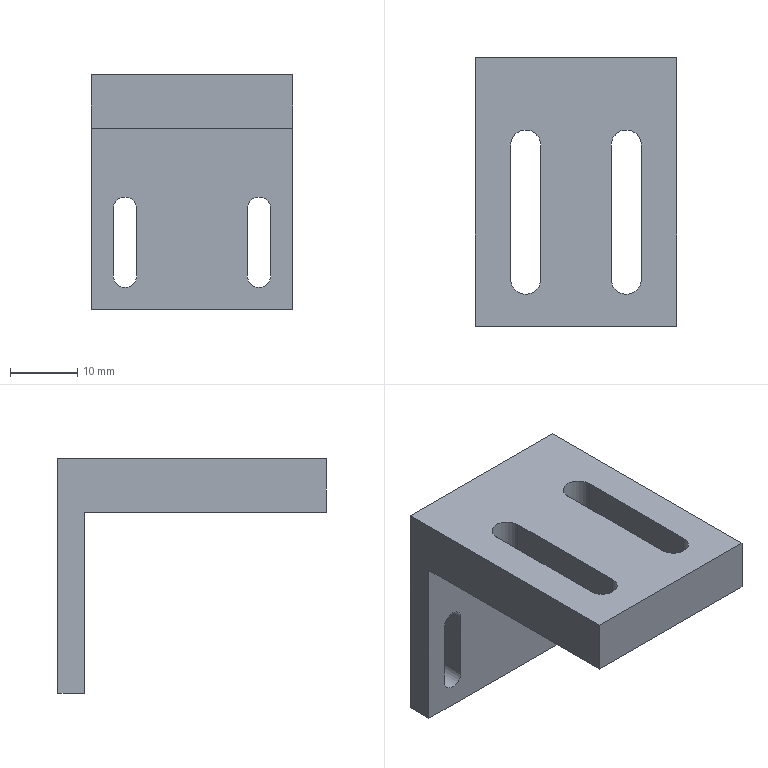Component | SolidWorks | CS021-A10-A028-1 | 1 solid | 26 faces | box 30 x 40 x 35 mm | volume 10789 mm3 | plane 16 | cylinder 10 | commonest cylinder face diameters 3.5 x6 4.5 x4 | material AL6061
build123d program:
from build123d import *

# Parameters (mm, degrees)
BOSS_EXTRUDE1_DEPTH = 15
CUT_EXTRUDE1_DEPTH  = 56.227
CUT_EXTRUDE2_DEPTH  = 56.227


with BuildPart() as part:
    # Sketch1 → Boss-Extrude1 (new, symmetric)
    with BuildSketch(Plane.XY):
        Polygon((0, 0), (8, 0), (8, 36), (35, 36), (35, 40), (0, 40), align=None)
    extrude(amount=BOSS_EXTRUDE1_DEPTH, both=True)

    # Sketch2 → Cut-Extrude1 (cut, through all)
    with BuildSketch(Plane.ZY):
        with BuildLine():
            Line((-9.75, 7), (-9.75, 27))
            ThreePointArc((-9.75, 27), (-7.5, 29.25), (-5.25, 27))
            Line((-5.25, 27), (-5.25, 7))
            ThreePointArc((-5.25, 7), (-7.5, 4.75), (-9.75, 7))
        make_face()
        with BuildLine():
            Line((9.75, 7), (9.75, 27))
            ThreePointArc((9.75, 27), (7.5, 29.25), (5.25, 27))
            Line((5.25, 27), (5.25, 7))
            ThreePointArc((5.25, 7), (7.5, 4.75), (9.75, 7))
        make_face()
    extrude(amount=-CUT_EXTRUDE1_DEPTH, mode=Mode.SUBTRACT)

    # Sketch3 → Cut-Extrude2 (cut, through all)
    with BuildSketch(Plane(origin=(0, 40, 0), x_dir=(1, 0, 0), z_dir=(0, 1, 0))):
        with BuildLine():
            Line((20, 11.75), (30, 11.75))
            ThreePointArc((30, 11.75), (31.75, 10), (30, 8.25))
            Line((30, 8.25), (20, 8.25))
            ThreePointArc((20, 8.25), (18.25, 10), (20, 11.75))
        make_face()
        with BuildLine():
            Line((20, -11.75), (30, -11.75))
            ThreePointArc((30, -11.75), (31.75, -10), (30, -8.25))
            Line((30, -8.25), (20, -8.25))
            ThreePointArc((20, -8.25), (18.25, -10), (20, -11.75))
        make_face()
    extrude(amount=-CUT_EXTRUDE2_DEPTH, mode=Mode.SUBTRACT)


solid = part.part

# Placed as in the assembly
solid = solid.moved(Location((152.449, 58.817, -55), (0, 90, 0)))
STEP:
#1=COLOUR_RGB('',0.7922,0.8196,0.9333);
#2=FILL_AREA_STYLE_COLOUR('',#1);
#3=FILL_AREA_STYLE('',(#2));
#4=SURFACE_STYLE_FILL_AREA(#3);
#5=SURFACE_SIDE_STYLE('',(#4));
#6=SURFACE_STYLE_USAGE(.BOTH.,#5);
#7=PRESENTATION_STYLE_ASSIGNMENT((#6));
#8=CARTESIAN_POINT('',(6.396,3.733,-2.884));
#9=VERTEX_POINT('',#8);
#10=CARTESIAN_POINT('',(6.465,3.733,-2.953));
#11=VERTEX_POINT('',#10);
#12=CARTESIAN_POINT('',(6.396,3.733,-2.953));
#13=DIRECTION('',(0.,1.,-0.));
#14=DIRECTION('',(1.,0.,0.));
#15=AXIS2_PLACEMENT_3D('',#12,#13,#14);
#16=CIRCLE('',#15,0.0689);
#17=EDGE_CURVE('',#9,#11,#16,.T.);
#18=ORIENTED_EDGE('',*,*,#17,.F.);
#19=CARTESIAN_POINT('',(6.396,3.89,-2.884));
#20=VERTEX_POINT('',#19);
#21=CARTESIAN_POINT('',(6.396,2.316,-2.884));
#22=DIRECTION('',(0.,1.,0.));
#23=VECTOR('',#22,39.37);
#24=LINE('',#21,#23);
#25=EDGE_CURVE('',#9,#20,#24,.T.);
#26=ORIENTED_EDGE('',*,*,#25,.T.);
#27=CARTESIAN_POINT('',(6.465,3.89,-2.953));
#28=VERTEX_POINT('',#27);
#29=CARTESIAN_POINT('',(6.396,3.89,-2.953));
#30=DIRECTION('',(0.,1.,0.));
#31=DIRECTION('',(0.,0.,-1.));
#32=AXIS2_PLACEMENT_3D('',#29,#30,#31);
#33=CIRCLE('',#32,0.0689);
#34=EDGE_CURVE('',#20,#28,#33,.T.);
#35=ORIENTED_EDGE('',*,*,#34,.T.);
#36=CARTESIAN_POINT('',(6.465,2.316,-2.953));
#37=DIRECTION('',(0.,1.,0.));
#38=VECTOR('',#37,39.37);
#39=LINE('',#36,#38);
#40=EDGE_CURVE('',#11,#28,#39,.T.);
#41=ORIENTED_EDGE('',*,*,#40,.F.);
#42=EDGE_LOOP('',(#18,#26,#35,#41));
#43=FACE_OUTER_BOUND('',#42,.T.);
#44=CARTESIAN_POINT('',(6.396,2.316,-2.953));
#45=DIRECTION('',(0.,1.,0.));
#46=DIRECTION('',(0.,0.,1.));
#47=AXIS2_PLACEMENT_3D('',#44,#45,#46);
#48=CYLINDRICAL_SURFACE('',#47,0.0689);
#49=ADVANCED_FACE('',(#43),#48,.F.);
#50=CARTESIAN_POINT('',(5.608,3.733,-2.884));
#51=VERTEX_POINT('',#50);
#52=CARTESIAN_POINT('',(5.677,3.733,-2.953));
#53=VERTEX_POINT('',#52);
#54=CARTESIAN_POINT('',(5.608,3.733,-2.953));
#55=DIRECTION('',(0.,1.,-0.));
#56=DIRECTION('',(1.,0.,0.));
#57=AXIS2_PLACEMENT_3D('',#54,#55,#56);
#58=CIRCLE('',#57,0.0689);
#59=EDGE_CURVE('',#51,#53,#58,.T.);
#60=ORIENTED_EDGE('',*,*,#59,.F.);
#61=CARTESIAN_POINT('',(5.608,3.89,-2.884));
#62=VERTEX_POINT('',#61);
#63=CARTESIAN_POINT('',(5.608,2.316,-2.884));
#64=DIRECTION('',(0.,1.,0.));
#65=VECTOR('',#64,39.37);
#66=LINE('',#63,#65);
#67=EDGE_CURVE('',#51,#62,#66,.T.);
#68=ORIENTED_EDGE('',*,*,#67,.T.);
#69=CARTESIAN_POINT('',(5.677,3.89,-2.953));
#70=VERTEX_POINT('',#69);
#71=CARTESIAN_POINT('',(5.608,3.89,-2.953));
#72=DIRECTION('',(0.,1.,0.));
#73=DIRECTION('',(0.,0.,1.));
#74=AXIS2_PLACEMENT_3D('',#71,#72,#73);
#75=CIRCLE('',#74,0.0689);
#76=EDGE_CURVE('',#62,#70,#75,.T.);
#77=ORIENTED_EDGE('',*,*,#76,.T.);
#78=CARTESIAN_POINT('',(5.677,2.316,-2.953));
#79=DIRECTION('',(0.,1.,0.));
#80=VECTOR('',#79,39.37);
#81=LINE('',#78,#80);
#82=EDGE_CURVE('',#53,#70,#81,.T.);
#83=ORIENTED_EDGE('',*,*,#82,.F.);
#84=EDGE_LOOP('',(#60,#68,#77,#83));
#85=FACE_OUTER_BOUND('',#84,.T.);
#86=CARTESIAN_POINT('',(5.608,2.316,-2.953));
#87=DIRECTION('',(0.,1.,0.));
#88=DIRECTION('',(0.,0.,1.));
#89=AXIS2_PLACEMENT_3D('',#86,#87,#88);
#90=CYLINDRICAL_SURFACE('',#89,0.0689);
#91=ADVANCED_FACE('',(#85),#90,.F.);
#92=CARTESIAN_POINT('',(6.386,2.591,-2.165));
#93=VERTEX_POINT('',#92);
#94=CARTESIAN_POINT('',(6.386,3.379,-2.165));
#95=VERTEX_POINT('',#94);
#96=CARTESIAN_POINT('',(6.386,2.591,-2.165));
#97=DIRECTION('',(0.,1.,-0.));
#98=VECTOR('',#97,39.37);
#99=LINE('',#96,#98);
#100=EDGE_CURVE('',#93,#95,#99,.T.);
#101=ORIENTED_EDGE('',*,*,#100,.F.);
#102=CARTESIAN_POINT('',(6.209,2.591,-2.165));
#103=VERTEX_POINT('',#102);
#104=CARTESIAN_POINT('',(6.297,2.591,-2.165));
#105=DIRECTION('',(0.,0.,1.));
#106=DIRECTION('',(-1.,0.,0.));
#107=AXIS2_PLACEMENT_3D('',#104,#105,#106);
#108=CIRCLE('',#107,0.08858);
#109=EDGE_CURVE('',#103,#93,#108,.T.);
#110=ORIENTED_EDGE('',*,*,#109,.F.);
#111=CARTESIAN_POINT('',(6.209,3.379,-2.165));
#112=VERTEX_POINT('',#111);
#113=CARTESIAN_POINT('',(6.209,2.591,-2.165));
#114=DIRECTION('',(-0.,-1.,0.));
#115=VECTOR('',#114,39.37);
#116=LINE('',#113,#115);
#117=EDGE_CURVE('',#112,#103,#116,.T.);
#118=ORIENTED_EDGE('',*,*,#117,.F.);
#119=CARTESIAN_POINT('',(6.297,3.379,-2.165));
#120=DIRECTION('',(0.,0.,1.));
#121=DIRECTION('',(-1.,0.,0.));
#122=AXIS2_PLACEMENT_3D('',#119,#120,#121);
#123=CIRCLE('',#122,0.08858);
#124=EDGE_CURVE('',#95,#112,#123,.T.);
#125=ORIENTED_EDGE('',*,*,#124,.F.);
#126=EDGE_LOOP('',(#101,#110,#118,#125));
#127=FACE_BOUND('',#126,.T.);
#128=CARTESIAN_POINT('',(5.795,2.591,-2.165));
#129=VERTEX_POINT('',#128);
#130=CARTESIAN_POINT('',(5.795,3.379,-2.165));
#131=VERTEX_POINT('',#130);
#132=CARTESIAN_POINT('',(5.795,2.591,-2.165));
#133=DIRECTION('',(0.,1.,-0.));
#134=VECTOR('',#133,39.37);
#135=LINE('',#132,#134);
#136=EDGE_CURVE('',#129,#131,#135,.T.);
#137=ORIENTED_EDGE('',*,*,#136,.F.);
#138=CARTESIAN_POINT('',(5.618,2.591,-2.165));
#139=VERTEX_POINT('',#138);
#140=CARTESIAN_POINT('',(5.707,2.591,-2.165));
#141=DIRECTION('',(0.,0.,1.));
#142=DIRECTION('',(1.,0.,0.));
#143=AXIS2_PLACEMENT_3D('',#140,#141,#142);
#144=CIRCLE('',#143,0.08858);
#145=EDGE_CURVE('',#139,#129,#144,.T.);
#146=ORIENTED_EDGE('',*,*,#145,.F.);
#147=CARTESIAN_POINT('',(5.618,3.379,-2.165));
#148=VERTEX_POINT('',#147);
#149=CARTESIAN_POINT('',(5.618,2.591,-2.165));
#150=DIRECTION('',(-0.,-1.,0.));
#151=VECTOR('',#150,39.37);
#152=LINE('',#149,#151);
#153=EDGE_CURVE('',#148,#139,#152,.T.);
#154=ORIENTED_EDGE('',*,*,#153,.F.);
#155=CARTESIAN_POINT('',(5.707,3.379,-2.165));
#156=DIRECTION('',(0.,0.,1.));
#157=DIRECTION('',(1.,0.,0.));
#158=AXIS2_PLACEMENT_3D('',#155,#156,#157);
#159=CIRCLE('',#158,0.08858);
#160=EDGE_CURVE('',#131,#148,#159,.T.);
#161=ORIENTED_EDGE('',*,*,#160,.F.);
#162=EDGE_LOOP('',(#137,#146,#154,#161));
#163=FACE_BOUND('',#162,.T.);
#164=CARTESIAN_POINT('',(5.411,3.89,-2.165));
#165=VERTEX_POINT('',#164);
#166=CARTESIAN_POINT('',(5.411,2.316,-2.165));
#167=VERTEX_POINT('',#166);
#168=CARTESIAN_POINT('',(5.411,3.89,-2.165));
#169=DIRECTION('',(-0.,-1.,0.));
#170=VECTOR('',#169,39.37);
#171=LINE('',#168,#170);
#172=EDGE_CURVE('',#165,#167,#171,.T.);
#173=ORIENTED_EDGE('',*,*,#172,.T.);
#174=CARTESIAN_POINT('',(6.592,2.316,-2.165));
#175=VERTEX_POINT('',#174);
#176=CARTESIAN_POINT('',(6.592,2.316,-2.165));
#177=DIRECTION('',(-1.,0.,0.));
#178=VECTOR('',#177,39.37);
#179=LINE('',#176,#178);
#180=EDGE_CURVE('',#175,#167,#179,.T.);
#181=ORIENTED_EDGE('',*,*,#180,.F.);
#182=CARTESIAN_POINT('',(6.592,3.89,-2.165));
#183=VERTEX_POINT('',#182);
#184=CARTESIAN_POINT('',(6.592,3.89,-2.165));
#185=DIRECTION('',(-0.,-1.,0.));
#186=VECTOR('',#185,39.37);
#187=LINE('',#184,#186);
#188=EDGE_CURVE('',#183,#175,#187,.T.);
#189=ORIENTED_EDGE('',*,*,#188,.F.);
#190=CARTESIAN_POINT('',(6.592,3.89,-2.165));
#191=DIRECTION('',(-1.,0.,0.));
#192=VECTOR('',#191,39.37);
#193=LINE('',#190,#192);
#194=EDGE_CURVE('',#183,#165,#193,.T.);
#195=ORIENTED_EDGE('',*,*,#194,.T.);
#196=EDGE_LOOP('',(#173,#181,#189,#195));
#197=FACE_OUTER_BOUND('',#196,.T.);
#198=CARTESIAN_POINT('',(6.592,3.89,-2.165));
#199=DIRECTION('',(-0.,-0.,-1.));
#200=DIRECTION('',(-1.,0.,0.));
#201=AXIS2_PLACEMENT_3D('',#198,#199,#200);
#202=PLANE('',#201);
#203=ADVANCED_FACE('',(#127,#163,#197),#202,.F.);
#204=CARTESIAN_POINT('',(5.411,2.316,-2.48));
#205=VERTEX_POINT('',#204);
#206=CARTESIAN_POINT('',(5.411,2.316,-2.165));
#207=DIRECTION('',(-0.,-0.,-1.));
#208=VECTOR('',#207,39.37);
#209=LINE('',#206,#208);
#210=EDGE_CURVE('',#167,#205,#209,.T.);
#211=ORIENTED_EDGE('',*,*,#210,.T.);
#212=CARTESIAN_POINT('',(6.592,2.316,-2.48));
#213=VERTEX_POINT('',#212);
#214=CARTESIAN_POINT('',(6.592,2.316,-2.48));
#215=DIRECTION('',(-1.,0.,0.));
#216=VECTOR('',#215,39.37);
#217=LINE('',#214,#216);
#218=EDGE_CURVE('',#213,#205,#217,.T.);
#219=ORIENTED_EDGE('',*,*,#218,.F.);
#220=CARTESIAN_POINT('',(6.592,2.316,-2.165));
#221=DIRECTION('',(-0.,-0.,-1.));
#222=VECTOR('',#221,39.37);
#223=LINE('',#220,#222);
#224=EDGE_CURVE('',#175,#213,#223,.T.);
#225=ORIENTED_EDGE('',*,*,#224,.F.);
#226=ORIENTED_EDGE('',*,*,#180,.T.);
#227=EDGE_LOOP('',(#211,#219,#225,#226));
#228=FACE_OUTER_BOUND('',#227,.T.);
#229=CARTESIAN_POINT('',(6.592,2.316,-2.165));
#230=DIRECTION('',(0.,1.,-0.));
#231=DIRECTION('',(1.,-0.,-0.));
#232=AXIS2_PLACEMENT_3D('',#229,#230,#231);
#233=PLANE('',#232);
#234=ADVANCED_FACE('',(#228),#233,.F.);
#235=CARTESIAN_POINT('',(6.209,3.379,-2.48));
#236=VERTEX_POINT('',#235);
#237=CARTESIAN_POINT('',(6.209,2.591,-2.48));
#238=VERTEX_POINT('',#237);
#239=CARTESIAN_POINT('',(6.209,2.316,-2.48));
#240=DIRECTION('',(-0.,-1.,0.));
#241=VECTOR('',#240,39.37);
#242=LINE('',#239,#241);
#243=EDGE_CURVE('',#236,#238,#242,.T.);
#244=ORIENTED_EDGE('',*,*,#243,.T.);
#245=CARTESIAN_POINT('',(6.386,2.591,-2.48));
#246=VERTEX_POINT('',#245);
#247=CARTESIAN_POINT('',(6.297,2.591,-2.48));
#248=DIRECTION('',(0.,0.,1.));
#249=DIRECTION('',(1.,0.,0.));
#250=AXIS2_PLACEMENT_3D('',#247,#248,#249);
#251=CIRCLE('',#250,0.08858);
#252=EDGE_CURVE('',#238,#246,#251,.T.);
#253=ORIENTED_EDGE('',*,*,#252,.T.);
#254=CARTESIAN_POINT('',(6.386,3.379,-2.48));
#255=VERTEX_POINT('',#254);
#256=CARTESIAN_POINT('',(6.386,2.316,-2.48));
#257=DIRECTION('',(0.,1.,-0.));
#258=VECTOR('',#257,39.37);
#259=LINE('',#256,#258);
#260=EDGE_CURVE('',#246,#255,#259,.T.);
#261=ORIENTED_EDGE('',*,*,#260,.T.);
#262=CARTESIAN_POINT('',(6.297,3.379,-2.48));
#263=DIRECTION('',(0.,0.,1.));
#264=DIRECTION('',(1.,0.,0.));
#265=AXIS2_PLACEMENT_3D('',#262,#263,#264);
#266=CIRCLE('',#265,0.08858);
#267=EDGE_CURVE('',#255,#236,#266,.T.);
#268=ORIENTED_EDGE('',*,*,#267,.T.);
#269=EDGE_LOOP('',(#244,#253,#261,#268));
#270=FACE_BOUND('',#269,.T.);
#271=CARTESIAN_POINT('',(5.618,3.379,-2.48));
#272=VERTEX_POINT('',#271);
#273=CARTESIAN_POINT('',(5.618,2.591,-2.48));
#274=VERTEX_POINT('',#273);
#275=CARTESIAN_POINT('',(5.618,2.316,-2.48));
#276=DIRECTION('',(-0.,-1.,0.));
#277=VECTOR('',#276,39.37);
#278=LINE('',#275,#277);
#279=EDGE_CURVE('',#272,#274,#278,.T.);
#280=ORIENTED_EDGE('',*,*,#279,.T.);
#281=CARTESIAN_POINT('',(5.795,2.591,-2.48));
#282=VERTEX_POINT('',#281);
#283=CARTESIAN_POINT('',(5.707,2.591,-2.48));
#284=DIRECTION('',(0.,0.,1.));
#285=DIRECTION('',(1.,0.,0.));
#286=AXIS2_PLACEMENT_3D('',#283,#284,#285);
#287=CIRCLE('',#286,0.08858);
#288=EDGE_CURVE('',#274,#282,#287,.T.);
#289=ORIENTED_EDGE('',*,*,#288,.T.);
#290=CARTESIAN_POINT('',(5.795,3.379,-2.48));
#291=VERTEX_POINT('',#290);
#292=CARTESIAN_POINT('',(5.795,2.316,-2.48));
#293=DIRECTION('',(0.,1.,-0.));
#294=VECTOR('',#293,39.37);
#295=LINE('',#292,#294);
#296=EDGE_CURVE('',#282,#291,#295,.T.);
#297=ORIENTED_EDGE('',*,*,#296,.T.);
#298=CARTESIAN_POINT('',(5.707,3.379,-2.48));
#299=DIRECTION('',(0.,0.,1.));
#300=DIRECTION('',(1.,0.,0.));
#301=AXIS2_PLACEMENT_3D('',#298,#299,#300);
#302=CIRCLE('',#301,0.08858);
#303=EDGE_CURVE('',#291,#272,#302,.T.);
#304=ORIENTED_EDGE('',*,*,#303,.T.);
#305=EDGE_LOOP('',(#280,#289,#297,#304));
#306=FACE_BOUND('',#305,.T.);
#307=CARTESIAN_POINT('',(5.411,3.733,-2.48));
#308=VERTEX_POINT('',#307);
#309=CARTESIAN_POINT('',(5.411,2.316,-2.48));
#310=DIRECTION('',(0.,1.,-0.));
#311=VECTOR('',#310,39.37);
#312=LINE('',#309,#311);
#313=EDGE_CURVE('',#205,#308,#312,.T.);
#314=ORIENTED_EDGE('',*,*,#313,.T.);
#315=CARTESIAN_POINT('',(6.592,3.733,-2.48));
#316=VERTEX_POINT('',#315);
#317=CARTESIAN_POINT('',(6.592,3.733,-2.48));
#318=DIRECTION('',(-1.,0.,0.));
#319=VECTOR('',#318,39.37);
#320=LINE('',#317,#319);
#321=EDGE_CURVE('',#316,#308,#320,.T.);
#322=ORIENTED_EDGE('',*,*,#321,.F.);
#323=CARTESIAN_POINT('',(6.592,2.316,-2.48));
#324=DIRECTION('',(0.,1.,-0.));
#325=VECTOR('',#324,39.37);
#326=LINE('',#323,#325);
#327=EDGE_CURVE('',#213,#316,#326,.T.);
#328=ORIENTED_EDGE('',*,*,#327,.F.);
#329=ORIENTED_EDGE('',*,*,#218,.T.);
#330=EDGE_LOOP('',(#314,#322,#328,#329));
#331=FACE_OUTER_BOUND('',#330,.T.);
#332=CARTESIAN_POINT('',(6.592,2.316,-2.48));
#333=DIRECTION('',(0.,0.,1.));
#334=DIRECTION('',(1.,-0.,-0.));
#335=AXIS2_PLACEMENT_3D('',#332,#333,#334);
#336=PLANE('',#335);
#337=ADVANCED_FACE('',(#270,#306,#331),#336,.F.);
#338=CARTESIAN_POINT('',(6.327,3.733,-3.346));
#339=VERTEX_POINT('',#338);
#340=CARTESIAN_POINT('',(6.327,3.733,-2.953));
#341=VERTEX_POINT('',#340);
#342=CARTESIAN_POINT('',(6.327,3.733,-2.48));
#343=DIRECTION('',(0.,0.,1.));
#344=VECTOR('',#343,39.37);
#345=LINE('',#342,#344);
#346=EDGE_CURVE('',#339,#341,#345,.T.);
#347=ORIENTED_EDGE('',*,*,#346,.T.);
#348=CARTESIAN_POINT('',(6.396,3.733,-2.953));
#349=DIRECTION('',(0.,1.,-0.));
#350=DIRECTION('',(1.,0.,0.));
#351=AXIS2_PLACEMENT_3D('',#348,#349,#350);
#352=CIRCLE('',#351,0.0689);
#353=EDGE_CURVE('',#341,#9,#352,.T.);
#354=ORIENTED_EDGE('',*,*,#353,.T.);
#355=ORIENTED_EDGE('',*,*,#17,.T.);
#356=CARTESIAN_POINT('',(6.465,3.733,-3.346));
#357=VERTEX_POINT('',#356);
#358=CARTESIAN_POINT('',(6.465,3.733,-2.48));
#359=DIRECTION('',(-0.,-0.,-1.));
#360=VECTOR('',#359,39.37);
#361=LINE('',#358,#360);
#362=EDGE_CURVE('',#11,#357,#361,.T.);
#363=ORIENTED_EDGE('',*,*,#362,.T.);
#364=CARTESIAN_POINT('',(6.396,3.733,-3.346));
#365=DIRECTION('',(0.,1.,-0.));
#366=DIRECTION('',(1.,0.,0.));
#367=AXIS2_PLACEMENT_3D('',#364,#365,#366);
#368=CIRCLE('',#367,0.0689);
#369=EDGE_CURVE('',#357,#339,#368,.T.);
#370=ORIENTED_EDGE('',*,*,#369,.T.);
#371=EDGE_LOOP('',(#347,#354,#355,#363,#370));
#372=FACE_BOUND('',#371,.T.);
#373=CARTESIAN_POINT('',(5.539,3.733,-3.346));
#374=VERTEX_POINT('',#373);
#375=CARTESIAN_POINT('',(5.539,3.733,-2.953));
#376=VERTEX_POINT('',#375);
#377=CARTESIAN_POINT('',(5.539,3.733,-2.48));
#378=DIRECTION('',(0.,0.,1.));
#379=VECTOR('',#378,39.37);
#380=LINE('',#377,#379);
#381=EDGE_CURVE('',#374,#376,#380,.T.);
#382=ORIENTED_EDGE('',*,*,#381,.T.);
#383=CARTESIAN_POINT('',(5.608,3.733,-2.953));
#384=DIRECTION('',(0.,1.,-0.));
#385=DIRECTION('',(1.,0.,0.));
#386=AXIS2_PLACEMENT_3D('',#383,#384,#385);
#387=CIRCLE('',#386,0.0689);
#388=EDGE_CURVE('',#376,#51,#387,.T.);
#389=ORIENTED_EDGE('',*,*,#388,.T.);
#390=ORIENTED_EDGE('',*,*,#59,.T.);
#391=CARTESIAN_POINT('',(5.677,3.733,-3.346));
#392=VERTEX_POINT('',#391);
#393=CARTESIAN_POINT('',(5.677,3.733,-2.48));
#394=DIRECTION('',(-0.,-0.,-1.));
#395=VECTOR('',#394,39.37);
#396=LINE('',#393,#395);
#397=EDGE_CURVE('',#53,#392,#396,.T.);
#398=ORIENTED_EDGE('',*,*,#397,.T.);
#399=CARTESIAN_POINT('',(5.608,3.733,-3.346));
#400=DIRECTION('',(0.,1.,-0.));
#401=DIRECTION('',(1.,0.,0.));
#402=AXIS2_PLACEMENT_3D('',#399,#400,#401);
#403=CIRCLE('',#402,0.0689);
#404=EDGE_CURVE('',#392,#374,#403,.T.);
#405=ORIENTED_EDGE('',*,*,#404,.T.);
#406=EDGE_LOOP('',(#382,#389,#390,#398,#405));
#407=FACE_BOUND('',#406,.T.);
#408=CARTESIAN_POINT('',(5.411,3.733,-3.543));
#409=VERTEX_POINT('',#408);
#410=CARTESIAN_POINT('',(5.411,3.733,-2.48));
#411=DIRECTION('',(-0.,-0.,-1.));
#412=VECTOR('',#411,39.37);
#413=LINE('',#410,#412);
#414=EDGE_CURVE('',#308,#409,#413,.T.);
#415=ORIENTED_EDGE('',*,*,#414,.T.);
#416=CARTESIAN_POINT('',(6.592,3.733,-3.543));
#417=VERTEX_POINT('',#416);
#418=CARTESIAN_POINT('',(6.592,3.733,-3.543));
#419=DIRECTION('',(-1.,0.,0.));
#420=VECTOR('',#419,39.37);
#421=LINE('',#418,#420);
#422=EDGE_CURVE('',#417,#409,#421,.T.);
#423=ORIENTED_EDGE('',*,*,#422,.F.);
#424=CARTESIAN_POINT('',(6.592,3.733,-2.48));
#425=DIRECTION('',(-0.,-0.,-1.));
#426=VECTOR('',#425,39.37);
#427=LINE('',#424,#426);
#428=EDGE_CURVE('',#316,#417,#427,.T.);
#429=ORIENTED_EDGE('',*,*,#428,.F.);
#430=ORIENTED_EDGE('',*,*,#321,.T.);
#431=EDGE_LOOP('',(#415,#423,#429,#430));
#432=FACE_OUTER_BOUND('',#431,.T.);
#433=CARTESIAN_POINT('',(6.592,3.733,-2.48));
#434=DIRECTION('',(0.,1.,-0.));
#435=DIRECTION('',(1.,-0.,-0.));
#436=AXIS2_PLACEMENT_3D('',#433,#434,#435);
#437=PLANE('',#436);
#438=ADVANCED_FACE('',(#372,#407,#432),#437,.F.);
#439=CARTESIAN_POINT('',(5.411,3.89,-3.543));
#440=VERTEX_POINT('',#439);
#441=CARTESIAN_POINT('',(5.411,3.733,-3.543));
#442=DIRECTION('',(0.,1.,-0.));
#443=VECTOR('',#442,39.37);
#444=LINE('',#441,#443);
#445=EDGE_CURVE('',#409,#440,#444,.T.);
#446=ORIENTED_EDGE('',*,*,#445,.T.);
#447=CARTESIAN_POINT('',(6.592,3.89,-3.543));
#448=VERTEX_POINT('',#447);
#449=CARTESIAN_POINT('',(6.592,3.89,-3.543));
#450=DIRECTION('',(-1.,0.,0.));
#451=VECTOR('',#450,39.37);
#452=LINE('',#449,#451);
#453=EDGE_CURVE('',#448,#440,#452,.T.);
#454=ORIENTED_EDGE('',*,*,#453,.F.);
#455=CARTESIAN_POINT('',(6.592,3.733,-3.543));
#456=DIRECTION('',(0.,1.,-0.));
#457=VECTOR('',#456,39.37);
#458=LINE('',#455,#457);
#459=EDGE_CURVE('',#417,#448,#458,.T.);
#460=ORIENTED_EDGE('',*,*,#459,.F.);
#461=ORIENTED_EDGE('',*,*,#422,.T.);
#462=EDGE_LOOP('',(#446,#454,#460,#461));
#463=FACE_OUTER_BOUND('',#462,.T.);
#464=CARTESIAN_POINT('',(6.592,3.733,-3.543));
#465=DIRECTION('',(0.,0.,1.));
#466=DIRECTION('',(1.,-0.,-0.));
#467=AXIS2_PLACEMENT_3D('',#464,#465,#466);
#468=PLANE('',#467);
#469=ADVANCED_FACE('',(#463),#468,.F.);
#470=CARTESIAN_POINT('',(6.465,3.89,-3.346));
#471=VERTEX_POINT('',#470);
#472=CARTESIAN_POINT('',(6.465,3.89,-2.953));
#473=DIRECTION('',(-0.,-0.,-1.));
#474=VECTOR('',#473,39.37);
#475=LINE('',#472,#474);
#476=EDGE_CURVE('',#28,#471,#475,.T.);
#477=ORIENTED_EDGE('',*,*,#476,.F.);
#478=ORIENTED_EDGE('',*,*,#34,.F.);
#479=CARTESIAN_POINT('',(6.327,3.89,-2.953));
#480=VERTEX_POINT('',#479);
#481=CARTESIAN_POINT('',(6.396,3.89,-2.953));
#482=DIRECTION('',(0.,1.,0.));
#483=DIRECTION('',(0.,0.,-1.));
#484=AXIS2_PLACEMENT_3D('',#481,#482,#483);
#485=CIRCLE('',#484,0.0689);
#486=EDGE_CURVE('',#480,#20,#485,.T.);
#487=ORIENTED_EDGE('',*,*,#486,.F.);
#488=CARTESIAN_POINT('',(6.327,3.89,-3.346));
#489=VERTEX_POINT('',#488);
#490=CARTESIAN_POINT('',(6.327,3.89,-2.953));
#491=DIRECTION('',(0.,0.,1.));
#492=VECTOR('',#491,39.37);
#493=LINE('',#490,#492);
#494=EDGE_CURVE('',#489,#480,#493,.T.);
#495=ORIENTED_EDGE('',*,*,#494,.F.);
#496=CARTESIAN_POINT('',(6.396,3.89,-3.346));
#497=DIRECTION('',(0.,1.,0.));
#498=DIRECTION('',(0.,0.,-1.));
#499=AXIS2_PLACEMENT_3D('',#496,#497,#498);
#500=CIRCLE('',#499,0.0689);
#501=EDGE_CURVE('',#471,#489,#500,.T.);
#502=ORIENTED_EDGE('',*,*,#501,.F.);
#503=EDGE_LOOP('',(#477,#478,#487,#495,#502));
#504=FACE_BOUND('',#503,.T.);
#505=CARTESIAN_POINT('',(5.677,3.89,-3.346));
#506=VERTEX_POINT('',#505);
#507=CARTESIAN_POINT('',(5.677,3.89,-2.953));
#508=DIRECTION('',(-0.,-0.,-1.));
#509=VECTOR('',#508,39.37);
#510=LINE('',#507,#509);
#511=EDGE_CURVE('',#70,#506,#510,.T.);
#512=ORIENTED_EDGE('',*,*,#511,.F.);
#513=ORIENTED_EDGE('',*,*,#76,.F.);
#514=CARTESIAN_POINT('',(5.539,3.89,-2.953));
#515=VERTEX_POINT('',#514);
#516=CARTESIAN_POINT('',(5.608,3.89,-2.953));
#517=DIRECTION('',(0.,1.,0.));
#518=DIRECTION('',(0.,0.,1.));
#519=AXIS2_PLACEMENT_3D('',#516,#517,#518);
#520=CIRCLE('',#519,0.0689);
#521=EDGE_CURVE('',#515,#62,#520,.T.);
#522=ORIENTED_EDGE('',*,*,#521,.F.);
#523=CARTESIAN_POINT('',(5.539,3.89,-3.346));
#524=VERTEX_POINT('',#523);
#525=CARTESIAN_POINT('',(5.539,3.89,-2.953));
#526=DIRECTION('',(0.,0.,1.));
#527=VECTOR('',#526,39.37);
#528=LINE('',#525,#527);
#529=EDGE_CURVE('',#524,#515,#528,.T.);
#530=ORIENTED_EDGE('',*,*,#529,.F.);
#531=CARTESIAN_POINT('',(5.608,3.89,-3.346));
#532=DIRECTION('',(0.,1.,0.));
#533=DIRECTION('',(0.,0.,1.));
#534=AXIS2_PLACEMENT_3D('',#531,#532,#533);
#535=CIRCLE('',#534,0.0689);
#536=EDGE_CURVE('',#506,#524,#535,.T.);
#537=ORIENTED_EDGE('',*,*,#536,.F.);
#538=EDGE_LOOP('',(#512,#513,#522,#530,#537));
#539=FACE_BOUND('',#538,.T.);
#540=CARTESIAN_POINT('',(5.411,3.89,-3.543));
#541=DIRECTION('',(0.,-0.,1.));
#542=VECTOR('',#541,39.37);
#543=LINE('',#540,#542);
#544=EDGE_CURVE('',#440,#165,#543,.T.);
#545=ORIENTED_EDGE('',*,*,#544,.T.);
#546=ORIENTED_EDGE('',*,*,#194,.F.);
#547=CARTESIAN_POINT('',(6.592,3.89,-3.543));
#548=DIRECTION('',(0.,-0.,1.));
#549=VECTOR('',#548,39.37);
#550=LINE('',#547,#549);
#551=EDGE_CURVE('',#448,#183,#550,.T.);
#552=ORIENTED_EDGE('',*,*,#551,.F.);
#553=ORIENTED_EDGE('',*,*,#453,.T.);
#554=EDGE_LOOP('',(#545,#546,#552,#553));
#555=FACE_OUTER_BOUND('',#554,.T.);
#556=CARTESIAN_POINT('',(6.592,3.89,-3.543));
#557=DIRECTION('',(-0.,-1.,-0.));
#558=DIRECTION('',(-0.,0.,-1.));
#559=AXIS2_PLACEMENT_3D('',#556,#557,#558);
#560=PLANE('',#559);
#561=ADVANCED_FACE('',(#504,#539,#555),#560,.F.);
#562=ORIENTED_EDGE('',*,*,#188,.T.);
#563=ORIENTED_EDGE('',*,*,#224,.T.);
#564=ORIENTED_EDGE('',*,*,#327,.T.);
#565=ORIENTED_EDGE('',*,*,#428,.T.);
#566=ORIENTED_EDGE('',*,*,#459,.T.);
#567=ORIENTED_EDGE('',*,*,#551,.T.);
#568=EDGE_LOOP('',(#562,#563,#564,#565,#566,#567));
#569=FACE_OUTER_BOUND('',#568,.T.);
#570=CARTESIAN_POINT('',(6.592,2.316,-2.165));
#571=DIRECTION('',(1.,-0.,-0.));
#572=DIRECTION('',(-0.,-0.,-1.));
#573=AXIS2_PLACEMENT_3D('',#570,#571,#572);
#574=PLANE('',#573);
#575=ADVANCED_FACE('',(#569),#574,.T.);
#576=ORIENTED_EDGE('',*,*,#172,.F.);
#577=ORIENTED_EDGE('',*,*,#544,.F.);
#578=ORIENTED_EDGE('',*,*,#445,.F.);
#579=ORIENTED_EDGE('',*,*,#414,.F.);
#580=ORIENTED_EDGE('',*,*,#313,.F.);
#581=ORIENTED_EDGE('',*,*,#210,.F.);
#582=EDGE_LOOP('',(#576,#577,#578,#579,#580,#581));
#583=FACE_OUTER_BOUND('',#582,.T.);
#584=CARTESIAN_POINT('',(5.411,2.316,-2.165));
#585=DIRECTION('',(1.,-0.,-0.));
#586=DIRECTION('',(-0.,-0.,-1.));
#587=AXIS2_PLACEMENT_3D('',#584,#585,#586);
#588=PLANE('',#587);
#589=ADVANCED_FACE('',(#583),#588,.F.);
#590=CARTESIAN_POINT('',(5.618,2.591,-3.543));
#591=DIRECTION('',(0.,0.,1.));
#592=VECTOR('',#591,39.37);
#593=LINE('',#590,#592);
#594=EDGE_CURVE('',#274,#139,#593,.T.);
#595=ORIENTED_EDGE('',*,*,#594,.T.);
#596=ORIENTED_EDGE('',*,*,#145,.T.);
#597=CARTESIAN_POINT('',(5.795,2.591,-3.543));
#598=DIRECTION('',(0.,0.,1.));
#599=VECTOR('',#598,39.37);
#600=LINE('',#597,#599);
#601=EDGE_CURVE('',#282,#129,#600,.T.);
#602=ORIENTED_EDGE('',*,*,#601,.F.);
#603=ORIENTED_EDGE('',*,*,#288,.F.);
#604=EDGE_LOOP('',(#595,#596,#602,#603));
#605=FACE_OUTER_BOUND('',#604,.T.);
#606=CARTESIAN_POINT('',(5.707,2.591,-3.543));
#607=DIRECTION('',(0.,0.,1.));
#608=DIRECTION('',(1.,0.,0.));
#609=AXIS2_PLACEMENT_3D('',#606,#607,#608);
#610=CYLINDRICAL_SURFACE('',#609,0.08858);
#611=ADVANCED_FACE('',(#605),#610,.F.);
#612=CARTESIAN_POINT('',(5.618,3.379,-3.543));
#613=DIRECTION('',(0.,0.,1.));
#614=VECTOR('',#613,39.37);
#615=LINE('',#612,#614);
#616=EDGE_CURVE('',#272,#148,#615,.T.);
#617=ORIENTED_EDGE('',*,*,#616,.T.);
#618=ORIENTED_EDGE('',*,*,#153,.T.);
#619=ORIENTED_EDGE('',*,*,#594,.F.);
#620=ORIENTED_EDGE('',*,*,#279,.F.);
#621=EDGE_LOOP('',(#617,#618,#619,#620));
#622=FACE_OUTER_BOUND('',#621,.T.);
#623=CARTESIAN_POINT('',(5.618,2.591,-3.543));
#624=DIRECTION('',(-1.,0.,0.));
#625=DIRECTION('',(0.,0.,1.));
#626=AXIS2_PLACEMENT_3D('',#623,#624,#625);
#627=PLANE('',#626);
#628=ADVANCED_FACE('',(#622),#627,.F.);
#629=CARTESIAN_POINT('',(5.795,3.379,-3.543));
#630=DIRECTION('',(0.,0.,1.));
#631=VECTOR('',#630,39.37);
#632=LINE('',#629,#631);
#633=EDGE_CURVE('',#291,#131,#632,.T.);
#634=ORIENTED_EDGE('',*,*,#633,.T.);
#635=ORIENTED_EDGE('',*,*,#160,.T.);
#636=ORIENTED_EDGE('',*,*,#616,.F.);
#637=ORIENTED_EDGE('',*,*,#303,.F.);
#638=EDGE_LOOP('',(#634,#635,#636,#637));
#639=FACE_OUTER_BOUND('',#638,.T.);
#640=CARTESIAN_POINT('',(5.707,3.379,-3.543));
#641=DIRECTION('',(0.,0.,1.));
#642=DIRECTION('',(1.,0.,0.));
#643=AXIS2_PLACEMENT_3D('',#640,#641,#642);
#644=CYLINDRICAL_SURFACE('',#643,0.08858);
#645=ADVANCED_FACE('',(#639),#644,.F.);
#646=ORIENTED_EDGE('',*,*,#601,.T.);
#647=ORIENTED_EDGE('',*,*,#136,.T.);
#648=ORIENTED_EDGE('',*,*,#633,.F.);
#649=ORIENTED_EDGE('',*,*,#296,.F.);
#650=EDGE_LOOP('',(#646,#647,#648,#649));
#651=FACE_OUTER_BOUND('',#650,.T.);
#652=CARTESIAN_POINT('',(5.795,2.591,-3.543));
#653=DIRECTION('',(1.,-0.,-0.));
#654=DIRECTION('',(-0.,-0.,-1.));
#655=AXIS2_PLACEMENT_3D('',#652,#653,#654);
#656=PLANE('',#655);
#657=ADVANCED_FACE('',(#651),#656,.F.);
#658=CARTESIAN_POINT('',(6.209,2.591,-3.543));
#659=DIRECTION('',(0.,0.,1.));
#660=VECTOR('',#659,39.37);
#661=LINE('',#658,#660);
#662=EDGE_CURVE('',#238,#103,#661,.T.);
#663=ORIENTED_EDGE('',*,*,#662,.T.);
#664=ORIENTED_EDGE('',*,*,#109,.T.);
#665=CARTESIAN_POINT('',(6.386,2.591,-3.543));
#666=DIRECTION('',(0.,0.,1.));
#667=VECTOR('',#666,39.37);
#668=LINE('',#665,#667);
#669=EDGE_CURVE('',#246,#93,#668,.T.);
#670=ORIENTED_EDGE('',*,*,#669,.F.);
#671=ORIENTED_EDGE('',*,*,#252,.F.);
#672=EDGE_LOOP('',(#663,#664,#670,#671));
#673=FACE_OUTER_BOUND('',#672,.T.);
#674=CARTESIAN_POINT('',(6.297,2.591,-3.543));
#675=DIRECTION('',(0.,0.,1.));
#676=DIRECTION('',(1.,0.,0.));
#677=AXIS2_PLACEMENT_3D('',#674,#675,#676);
#678=CYLINDRICAL_SURFACE('',#677,0.08858);
#679=ADVANCED_FACE('',(#673),#678,.F.);
#680=CARTESIAN_POINT('',(6.209,3.379,-3.543));
#681=DIRECTION('',(0.,0.,1.));
#682=VECTOR('',#681,39.37);
#683=LINE('',#680,#682);
#684=EDGE_CURVE('',#236,#112,#683,.T.);
#685=ORIENTED_EDGE('',*,*,#684,.T.);
#686=ORIENTED_EDGE('',*,*,#117,.T.);
#687=ORIENTED_EDGE('',*,*,#662,.F.);
#688=ORIENTED_EDGE('',*,*,#243,.F.);
#689=EDGE_LOOP('',(#685,#686,#687,#688));
#690=FACE_OUTER_BOUND('',#689,.T.);
#691=CARTESIAN_POINT('',(6.209,2.591,-3.543));
#692=DIRECTION('',(-1.,0.,0.));
#693=DIRECTION('',(0.,0.,1.));
#694=AXIS2_PLACEMENT_3D('',#691,#692,#693);
#695=PLANE('',#694);
#696=ADVANCED_FACE('',(#690),#695,.F.);
#697=CARTESIAN_POINT('',(6.386,3.379,-3.543));
#698=DIRECTION('',(0.,0.,1.));
#699=VECTOR('',#698,39.37);
#700=LINE('',#697,#699);
#701=EDGE_CURVE('',#255,#95,#700,.T.);
#702=ORIENTED_EDGE('',*,*,#701,.T.);
#703=ORIENTED_EDGE('',*,*,#124,.T.);
#704=ORIENTED_EDGE('',*,*,#684,.F.);
#705=ORIENTED_EDGE('',*,*,#267,.F.);
#706=EDGE_LOOP('',(#702,#703,#704,#705));
#707=FACE_OUTER_BOUND('',#706,.T.);
#708=CARTESIAN_POINT('',(6.297,3.379,-3.543));
#709=DIRECTION('',(0.,0.,1.));
#710=DIRECTION('',(1.,0.,0.));
#711=AXIS2_PLACEMENT_3D('',#708,#709,#710);
#712=CYLINDRICAL_SURFACE('',#711,0.08858);
#713=ADVANCED_FACE('',(#707),#712,.F.);
#714=ORIENTED_EDGE('',*,*,#669,.T.);
#715=ORIENTED_EDGE('',*,*,#100,.T.);
#716=ORIENTED_EDGE('',*,*,#701,.F.);
#717=ORIENTED_EDGE('',*,*,#260,.F.);
#718=EDGE_LOOP('',(#714,#715,#716,#717));
#719=FACE_OUTER_BOUND('',#718,.T.);
#720=CARTESIAN_POINT('',(6.386,2.591,-3.543));
#721=DIRECTION('',(1.,-0.,-0.));
#722=DIRECTION('',(-0.,-0.,-1.));
#723=AXIS2_PLACEMENT_3D('',#720,#721,#722);
#724=PLANE('',#723);
#725=ADVANCED_FACE('',(#719),#724,.F.);
#726=ORIENTED_EDGE('',*,*,#67,.F.);
#727=ORIENTED_EDGE('',*,*,#388,.F.);
#728=CARTESIAN_POINT('',(5.539,2.316,-2.953));
#729=DIRECTION('',(0.,1.,0.));
#730=VECTOR('',#729,39.37);
#731=LINE('',#728,#730);
#732=EDGE_CURVE('',#376,#515,#731,.T.);
#733=ORIENTED_EDGE('',*,*,#732,.T.);
#734=ORIENTED_EDGE('',*,*,#521,.T.);
#735=EDGE_LOOP('',(#726,#727,#733,#734));
#736=FACE_OUTER_BOUND('',#735,.T.);
#737=CARTESIAN_POINT('',(5.608,2.316,-2.953));
#738=DIRECTION('',(0.,1.,0.));
#739=DIRECTION('',(0.,0.,1.));
#740=AXIS2_PLACEMENT_3D('',#737,#738,#739);
#741=CYLINDRICAL_SURFACE('',#740,0.0689);
#742=ADVANCED_FACE('',(#736),#741,.F.);
#743=CARTESIAN_POINT('',(5.539,2.316,-3.346));
#744=DIRECTION('',(0.,1.,0.));
#745=VECTOR('',#744,39.37);
#746=LINE('',#743,#745);
#747=EDGE_CURVE('',#374,#524,#746,.T.);
#748=ORIENTED_EDGE('',*,*,#747,.T.);
#749=ORIENTED_EDGE('',*,*,#529,.T.);
#750=ORIENTED_EDGE('',*,*,#732,.F.);
#751=ORIENTED_EDGE('',*,*,#381,.F.);
#752=EDGE_LOOP('',(#748,#749,#750,#751));
#753=FACE_OUTER_BOUND('',#752,.T.);
#754=CARTESIAN_POINT('',(5.539,2.316,-2.953));
#755=DIRECTION('',(-1.,0.,0.));
#756=DIRECTION('',(0.,0.,1.));
#757=AXIS2_PLACEMENT_3D('',#754,#755,#756);
#758=PLANE('',#757);
#759=ADVANCED_FACE('',(#753),#758,.F.);
#760=CARTESIAN_POINT('',(5.677,2.316,-3.346));
#761=DIRECTION('',(0.,1.,0.));
#762=VECTOR('',#761,39.37);
#763=LINE('',#760,#762);
#764=EDGE_CURVE('',#392,#506,#763,.T.);
#765=ORIENTED_EDGE('',*,*,#764,.T.);
#766=ORIENTED_EDGE('',*,*,#536,.T.);
#767=ORIENTED_EDGE('',*,*,#747,.F.);
#768=ORIENTED_EDGE('',*,*,#404,.F.);
#769=EDGE_LOOP('',(#765,#766,#767,#768));
#770=FACE_OUTER_BOUND('',#769,.T.);
#771=CARTESIAN_POINT('',(5.608,2.316,-3.346));
#772=DIRECTION('',(0.,1.,0.));
#773=DIRECTION('',(0.,0.,1.));
#774=AXIS2_PLACEMENT_3D('',#771,#772,#773);
#775=CYLINDRICAL_SURFACE('',#774,0.0689);
#776=ADVANCED_FACE('',(#770),#775,.F.);
#777=ORIENTED_EDGE('',*,*,#82,.T.);
#778=ORIENTED_EDGE('',*,*,#511,.T.);
#779=ORIENTED_EDGE('',*,*,#764,.F.);
#780=ORIENTED_EDGE('',*,*,#397,.F.);
#781=EDGE_LOOP('',(#777,#778,#779,#780));
#782=FACE_OUTER_BOUND('',#781,.T.);
#783=CARTESIAN_POINT('',(5.677,2.316,-2.953));
#784=DIRECTION('',(1.,-0.,-0.));
#785=DIRECTION('',(-0.,-0.,-1.));
#786=AXIS2_PLACEMENT_3D('',#783,#784,#785);
#787=PLANE('',#786);
#788=ADVANCED_FACE('',(#782),#787,.F.);
#789=ORIENTED_EDGE('',*,*,#25,.F.);
#790=ORIENTED_EDGE('',*,*,#353,.F.);
#791=CARTESIAN_POINT('',(6.327,2.316,-2.953));
#792=DIRECTION('',(0.,1.,0.));
#793=VECTOR('',#792,39.37);
#794=LINE('',#791,#793);
#795=EDGE_CURVE('',#341,#480,#794,.T.);
#796=ORIENTED_EDGE('',*,*,#795,.T.);
#797=ORIENTED_EDGE('',*,*,#486,.T.);
#798=EDGE_LOOP('',(#789,#790,#796,#797));
#799=FACE_OUTER_BOUND('',#798,.T.);
#800=CARTESIAN_POINT('',(6.396,2.316,-2.953));
#801=DIRECTION('',(0.,1.,0.));
#802=DIRECTION('',(0.,0.,1.));
#803=AXIS2_PLACEMENT_3D('',#800,#801,#802);
#804=CYLINDRICAL_SURFACE('',#803,0.0689);
#805=ADVANCED_FACE('',(#799),#804,.F.);
#806=CARTESIAN_POINT('',(6.327,2.316,-3.346));
#807=DIRECTION('',(0.,1.,0.));
#808=VECTOR('',#807,39.37);
#809=LINE('',#806,#808);
#810=EDGE_CURVE('',#339,#489,#809,.T.);
#811=ORIENTED_EDGE('',*,*,#810,.T.);
#812=ORIENTED_EDGE('',*,*,#494,.T.);
#813=ORIENTED_EDGE('',*,*,#795,.F.);
#814=ORIENTED_EDGE('',*,*,#346,.F.);
#815=EDGE_LOOP('',(#811,#812,#813,#814));
#816=FACE_OUTER_BOUND('',#815,.T.);
#817=CARTESIAN_POINT('',(6.327,2.316,-2.953));
#818=DIRECTION('',(-1.,0.,0.));
#819=DIRECTION('',(0.,0.,1.));
#820=AXIS2_PLACEMENT_3D('',#817,#818,#819);
#821=PLANE('',#820);
#822=ADVANCED_FACE('',(#816),#821,.F.);
#823=CARTESIAN_POINT('',(6.465,2.316,-3.346));
#824=DIRECTION('',(0.,1.,0.));
#825=VECTOR('',#824,39.37);
#826=LINE('',#823,#825);
#827=EDGE_CURVE('',#357,#471,#826,.T.);
#828=ORIENTED_EDGE('',*,*,#827,.T.);
#829=ORIENTED_EDGE('',*,*,#501,.T.);
#830=ORIENTED_EDGE('',*,*,#810,.F.);
#831=ORIENTED_EDGE('',*,*,#369,.F.);
#832=EDGE_LOOP('',(#828,#829,#830,#831));
#833=FACE_OUTER_BOUND('',#832,.T.);
#834=CARTESIAN_POINT('',(6.396,2.316,-3.346));
#835=DIRECTION('',(0.,1.,0.));
#836=DIRECTION('',(0.,0.,1.));
#837=AXIS2_PLACEMENT_3D('',#834,#835,#836);
#838=CYLINDRICAL_SURFACE('',#837,0.0689);
#839=ADVANCED_FACE('',(#833),#838,.F.);
#840=ORIENTED_EDGE('',*,*,#40,.T.);
#841=ORIENTED_EDGE('',*,*,#476,.T.);
#842=ORIENTED_EDGE('',*,*,#827,.F.);
#843=ORIENTED_EDGE('',*,*,#362,.F.);
#844=EDGE_LOOP('',(#840,#841,#842,#843));
#845=FACE_OUTER_BOUND('',#844,.T.);
#846=CARTESIAN_POINT('',(6.465,2.316,-2.953));
#847=DIRECTION('',(1.,-0.,-0.));
#848=DIRECTION('',(-0.,-0.,-1.));
#849=AXIS2_PLACEMENT_3D('',#846,#847,#848);
#850=PLANE('',#849);
#851=ADVANCED_FACE('',(#845),#850,.F.);
#852=CLOSED_SHELL('',(#49,#91,#203,#234,#337,#438,#469,#561,#575,#589,#611,#628,#645,#657,#679,#696,#713,#725,#742,#759,#776,#788,#805,#822,#839,#851));
#853=MANIFOLD_SOLID_BREP('',#852);
#854=STYLED_ITEM('',(#7),#853);
#855=(LENGTH_UNIT()NAMED_UNIT(*)SI_UNIT($,.METRE.));
#856=LENGTH_MEASURE_WITH_UNIT(LENGTH_MEASURE(0.0254),#855);
#857=DIMENSIONAL_EXPONENTS(1.,0.,0.,0.,0.,0.,0.);
#858=(CONVERSION_BASED_UNIT('',#856)LENGTH_UNIT()NAMED_UNIT(#857));
#859=UNCERTAINTY_MEASURE_WITH_UNIT(LENGTH_MEASURE(0.00001),#858,'','');
#860=(NAMED_UNIT(*)PLANE_ANGLE_UNIT()SI_UNIT($,.RADIAN.));
#861=(NAMED_UNIT(*)SI_UNIT($,.STERADIAN.)SOLID_ANGLE_UNIT());
#862=(GEOMETRIC_REPRESENTATION_CONTEXT(3)GLOBAL_UNCERTAINTY_ASSIGNED_CONTEXT((#859))GLOBAL_UNIT_ASSIGNED_CONTEXT((#858,#860,#861))REPRESENTATION_CONTEXT('',''));
#863=MECHANICAL_DESIGN_GEOMETRIC_PRESENTATION_REPRESENTATION('',(#854),#862);
#864=CARTESIAN_POINT('',(0.,0.,0.));
#865=DIRECTION('',(0.,0.,1.));
#866=DIRECTION('',(1.,0.,0.));
#867=AXIS2_PLACEMENT_3D('',#864,#865,#866);
#868=(LENGTH_UNIT()NAMED_UNIT(*)SI_UNIT($,.METRE.));
#869=LENGTH_MEASURE_WITH_UNIT(LENGTH_MEASURE(0.0254),#868);
#870=DIMENSIONAL_EXPONENTS(1.,0.,0.,0.,0.,0.,0.);
#871=(CONVERSION_BASED_UNIT('',#869)LENGTH_UNIT()NAMED_UNIT(#870));
#872=UNCERTAINTY_MEASURE_WITH_UNIT(LENGTH_MEASURE(0.00001),#871,'','');
#873=(NAMED_UNIT(*)PLANE_ANGLE_UNIT()SI_UNIT($,.RADIAN.));
#874=(NAMED_UNIT(*)SI_UNIT($,.STERADIAN.)SOLID_ANGLE_UNIT());
#875=(GEOMETRIC_REPRESENTATION_CONTEXT(3)GLOBAL_UNCERTAINTY_ASSIGNED_CONTEXT((#872))GLOBAL_UNIT_ASSIGNED_CONTEXT((#871,#873,#874))REPRESENTATION_CONTEXT('',''));
#876=ADVANCED_BREP_SHAPE_REPRESENTATION('',(#853,#867),#875);
#877=PRESENTATION_LAYER_ASSIGNMENT('','',(#854));